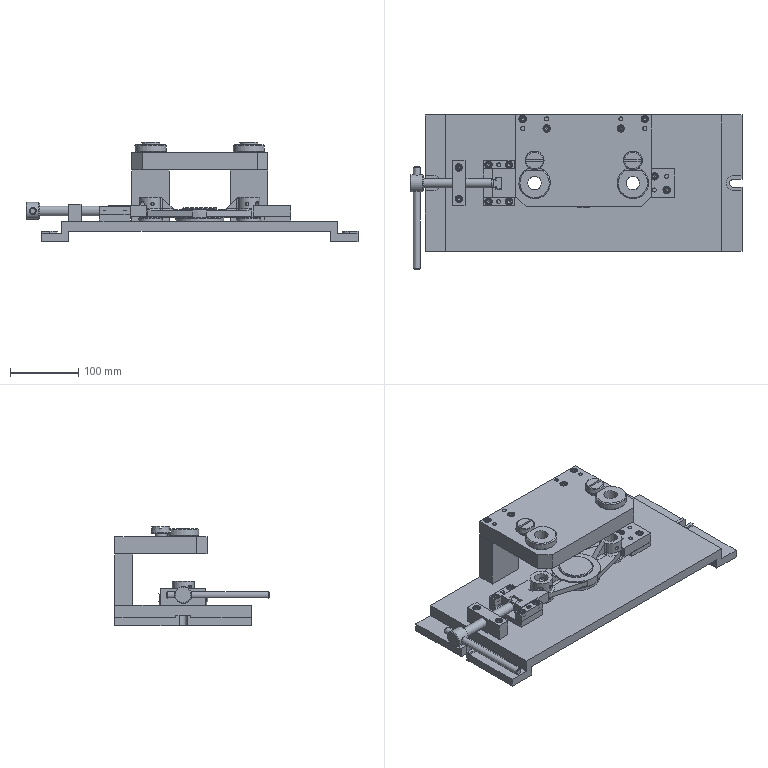Assembly | NX | mm | 37 component files | 37 solids | 739 faces | box 486.63 x 226 x 145.5 mm | volume 2611044 mm3 | plane 403 | cone 152 | cylinder 146 | torus 34 | sphere 4 | commonest cylinder face diameters 6 x44 10 x14 11 x13 5.795 x12 6.6 x12 35 x6 14 x6 8 x6
Bill of materials:
GB-T70.1-2000,M6x25 | 4 |  | Hexagon Socket Head Cap Screw, GB-T 70.1-2000,M6x25
unnamed part 1 | 1 |  | Long, slender solid cylindrical rod with small chamfers or edge breaks at both ends.
unnamed part 2 | 2 |  | Flanged cylindrical bushing with a through bore. One flat is cut into part of the flange edge. Short neck or groove under the flange, chamfered edges.
unnamed part 3 | 2 |  | Rectangular bar-shaped block with three vertical through-holes in a row: two larger holes at the ends and a smaller one in the middle.
GB-T119.1-2000,6x20 | 4 |  | Parallel Pin, GB-T 119.1-2000,6x20
unnamed part 4 | 2 |  | Slotted-head cylindrical fastener-like part: a round head with tapered sides and one straight slot across the top, a stepped collar under the head, and a smaller cylindrical shank with a chamfered end.
unnamed part 5 | 1 |  | Large rectangular base plate. It has stepped edge flanges and a U-shaped slot in the middle of each short end. Two tall rectangular blocks stand on top, with small holes in their top faces. There is also a central stepped cylindrical boss, two ring bosses with holes, two low pads with hole patterns, and several small holes.
unnamed part 6 | 1 |  | Rectangular block with a notch cut into one side, formed by angled faces leading to a rectangular slot, and four through-holes arranged in a 2x2 pattern.
GB-T70.1-2000,M6x16 | 6 |  | Hexagon Socket Head Cap Screw, GB-T 70.1-2000,M6x16
unnamed part 7 | 1 |  | Rectangular block with two vertical through-holes near its ends and one larger horizontal through-hole across the middle of its long side face.
unnamed part 8 | 2 |  | Thin-walled cylindrical tube or sleeve with plain square-cut ends.
GB-T70.1-2000,M6x30 | 2 |  | Hexagon Socket Head Cap Screw, GB-T 70.1-2000,M6x30
unnamed part 9 | 1 |  | Prismatic block with a rectangular slot cut into one end and, on the opposite end, a notch formed by angled faces leading to a rectangular slot.
unnamed part 10 | 1 |  | Rectangular flat plate with two chamfered corners. It has two large through-holes and two medium through-holes near the chamfered edge, and two 2x2 groups of small holes along the opposite edge.
GB-T119.1-2000,6x26 | 4 |  | Parallel Pin, GB-T 119.1-2000,6x26
unnamed part 11 | 1 |  | Stepped cylindrical pin with an enlarged cylindrical head pierced by a cross hole, a long main shank, and two smaller stepped diameters at the far end.
unnamed part 12 | 1 |  | Rectangular block with a large circular through-hole across its main side face and a rectangular step or tongue on one end, giving a T-shaped outline in plan.
unnamed part 13 | 1 |  | Symmetric flat, roughly diamond-shaped plate. It has a large circular through-hole in the middle, surrounded by a shallow raised ring. At each end of the long axis is a taller cylindrical boss with a vertical through-bore. Triangular gusset ribs join each boss to the plate. The bosses also have small radial cross-holes.
Mates:
1. fix | jig_body 1 component
2. concentric | workpiece 1 edge | jig_body 1 edge
3. touch align | workpiece 1 face | jig_body 1 face
4. touch align | V_block 1 face | workpiece 1 face
5. touch align | V_block 1 face | workpiece 1 face
6. parallel | V_block 1 face | jig_body 1 face
7. distance | jig_body 1 face | V_block 1 face
8. touch align | guide_block 2 face | jig_body 1 face
9. touch align | guide_block 2 face | jig_body 1 face
10. touch align | guide_block 2 face | jig_body 1 face
11. touch align | drill_template 1 face | workpiece 1 face
12. concentric | drill_bushing 2 edge | drill_template 1 edge
13. concentric | sleeve 2 edge | drill_template 1 edge
14. concentric | drill_template 1 edge | jig_body 1 edge
15. touch align | fixed_block 1 face | jig_body 1
16. concentric | fixed_block 1 edge | jig_body 1 arc
17. concentric | screw_rod 1 edge | stop_block 1 arc
18. touch align | screw_rod 1 face | fixed_block 1
19. touch align | stop_block 1 face | V_block 1 face
20. touch align | reamer_bar 1 face | screw_rod 1 face
21. concentric | drill_bushing_screw 2 edge | drill_template 1 arc
22. concentric | GB-T70_1-2000_M6x25 4 edge | drill_template 1 edge
23. concentric | GB-T70_1-2000_M6x25 3 edge | drill_template 1 edge
24. concentric | GB-T119_1-2000_6x26 4 edge | drill_template 1 edge
25. concentric | GB-T119_1-2000_6x26 3 edge | drill_template 1 edge
26. concentric | GB-T70_1-2000_M6x30 2 edge | fixed_block 1 edge
27. concentric | GB-T70_1-2000_M6x30 1 edge | fixed_block 1 edge
28. bond | guide_block 2 component | assembly component
29. bond | guide_block 2 component | assembly component
30. bond | guide_block 1 component | assembly component
31. linear | assembly datumaxis | assembly cartesiancoordinatesystem | assembly cartesiancoordinatesystem
32. concentric | GB-T119_1-2000_6x20 4 edge | guide_block 1 edge
33. concentric | GB-T70_1-2000_M6x16 6 edge | guide_block 1 edge
34. concentric | GB-T70_1-2000_M6x16 5 edge | guide_block 1 edge
35. bond | guide_block 2 component | assembly component
36. bond | GB-T70_1-2000_M6x16 6 component | assembly component
37. bond | GB-T119_1-2000_6x20 4 component | assembly component
38. bond | GB-T70_1-2000_M6x16 5 component | assembly component
39. bond | GB-T70_1-2000_M6x16 4 component | assembly component
40. bond | GB-T119_1-2000_6x20 3 component | assembly component
41. bond | GB-T70_1-2000_M6x16 3 component | assembly component
42. linear | assembly datumaxis | assembly cartesiancoordinatesystem | assembly cartesiancoordinatesystem
43. linear | assembly datumaxis | assembly cartesiancoordinatesystem | assembly cartesiancoordinatesystem
44. linear | assembly datumaxis | assembly cartesiancoordinatesystem | assembly cartesiancoordinatesystem
45. bond | drill_template 1 component | assembly component
46. bond | drill_bushing 2 component | assembly component
47. bond | sleeve 2 component | assembly component
48. bond | drill_bushing_screw 2 component | assembly component
49. bond | drill_bushing 1 component | assembly component
50. bond | sleeve 1 component | assembly component
51. bond | drill_bushing_screw 1 component | assembly component
52. linear | assembly datumaxis | assembly cartesiancoordinatesystem | assembly cartesiancoordinatesystem
53. linear | assembly datumaxis | assembly cartesiancoordinatesystem | assembly cartesiancoordinatesystem
54. linear | assembly datumaxis | assembly cartesiancoordinatesystem | assembly cartesiancoordinatesystem
55. touch align | fixed_V_block 1 face | jig_body 1
56. concentric | fixed_V_block 1 edge | jig_body 1 arc
57. concentric | GB-T70_1-2000_M6x16 1 edge | fixed_V_block 1 edge
58. concentric | GB-T70_1-2000_M6x16 2 edge | fixed_V_block 1 edge
59. concentric | GB-T119_1-2000_6x20 1 edge | fixed_V_block 1 edge
60. concentric | GB-T119_1-2000_6x20 2 edge | fixed_V_block 1 edge
61. concentric | GB-T70_1-2000_M6x25 2 edge | drill_template 1 edge
62. concentric | GB-T70_1-2000_M6x25 1 edge | drill_template 1 edge
63. concentric | GB-T119_1-2000_6x26 1 edge | drill_template 1 edge
64. concentric | GB-T119_1-2000_6x26 2 edge | drill_template 1 edge